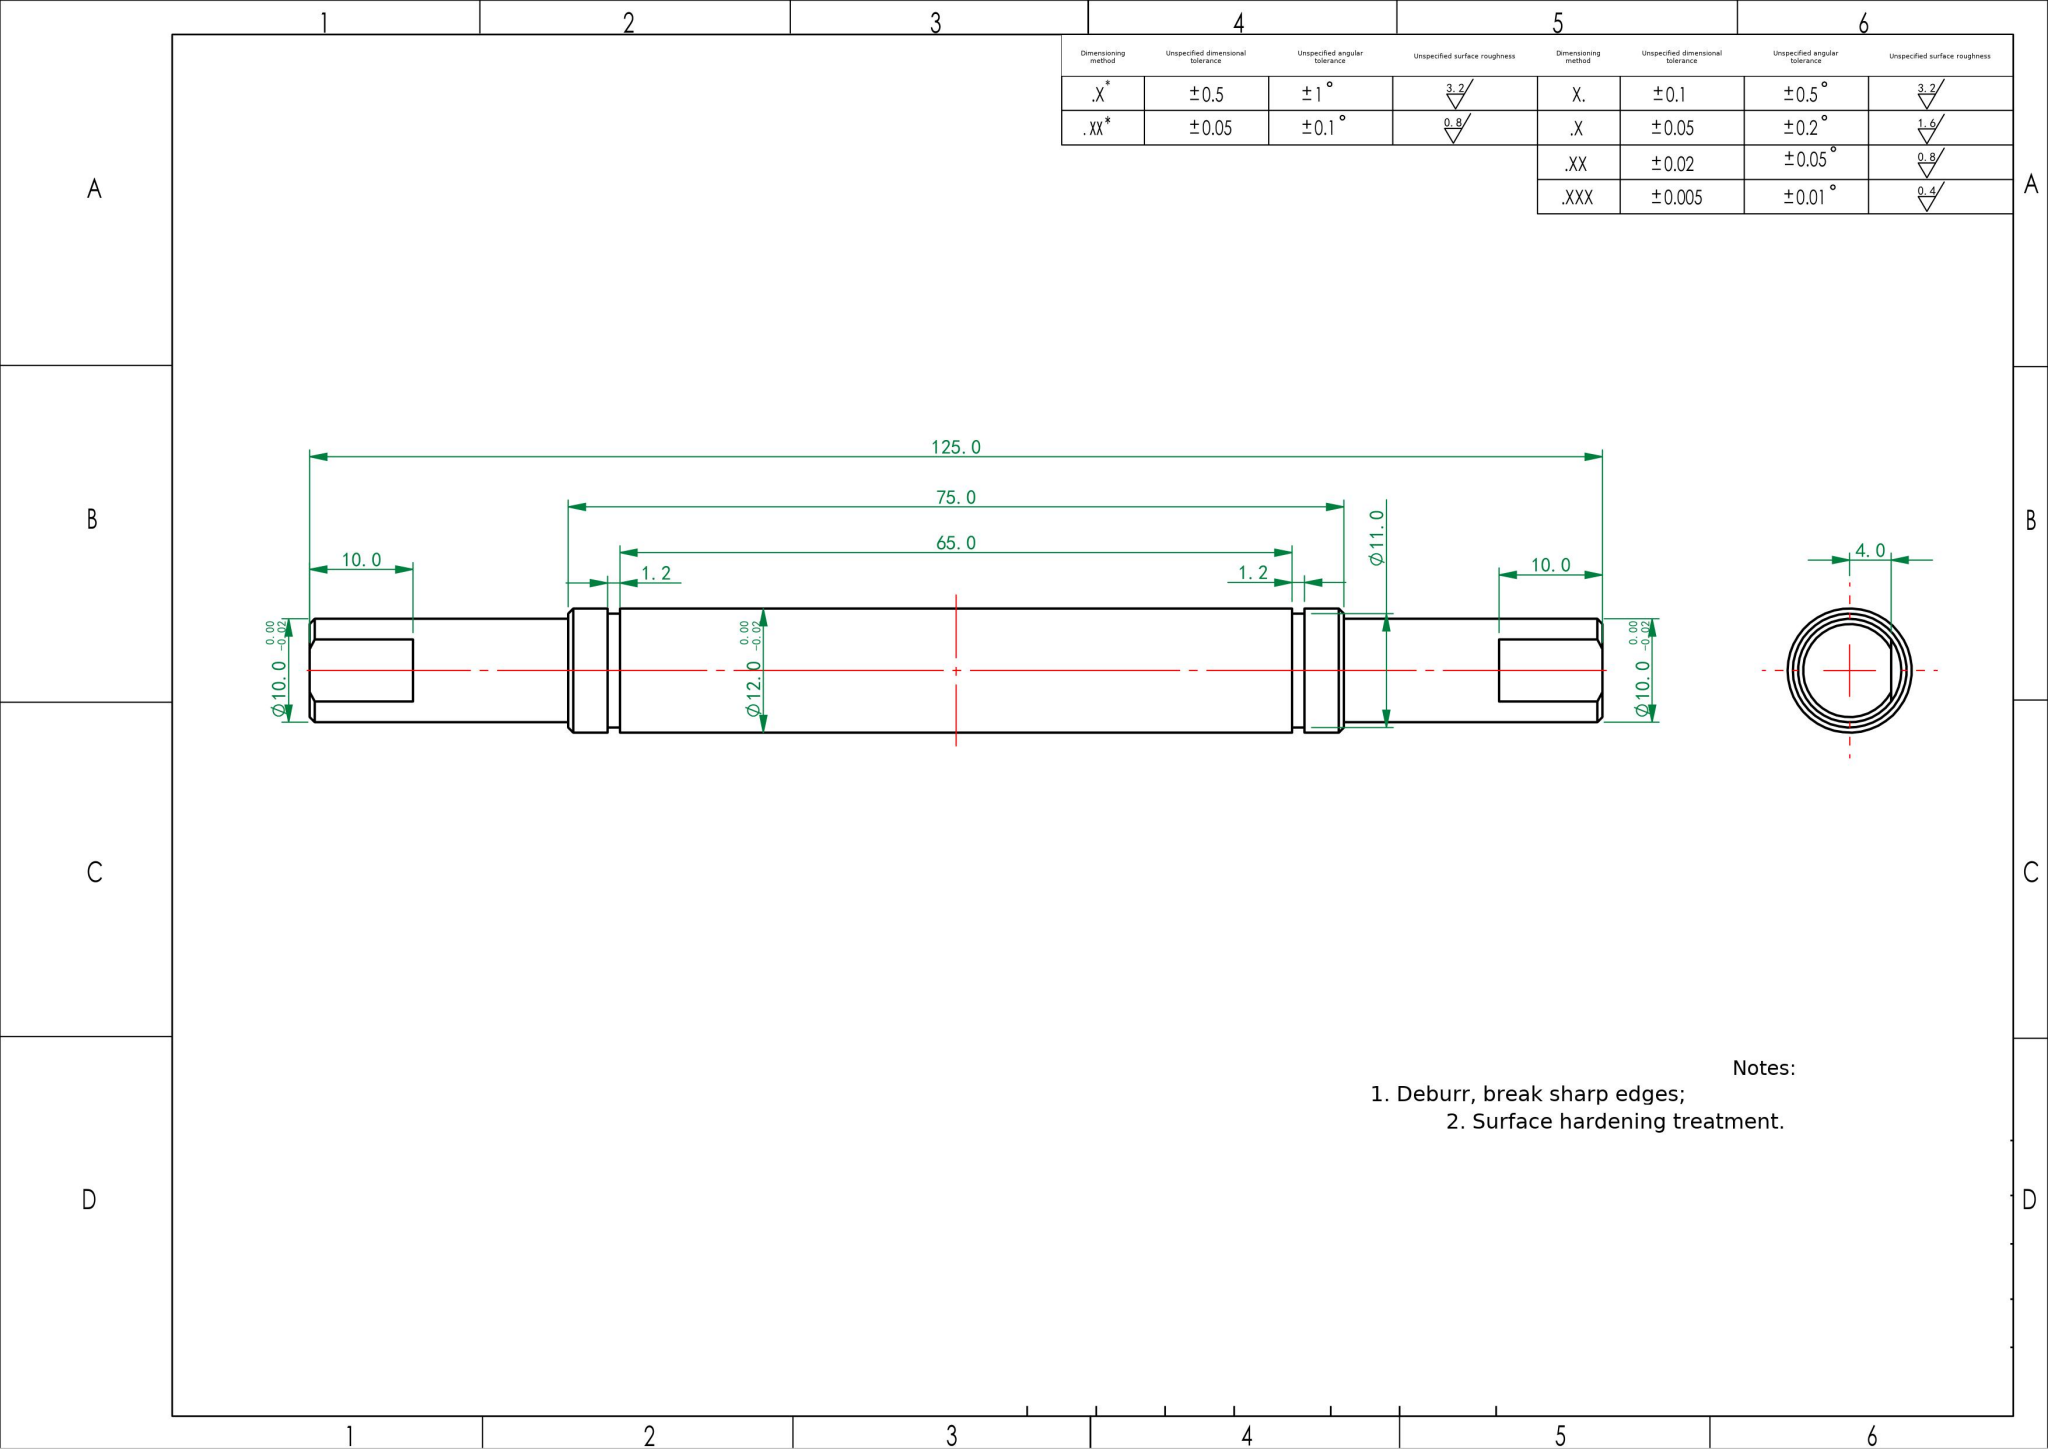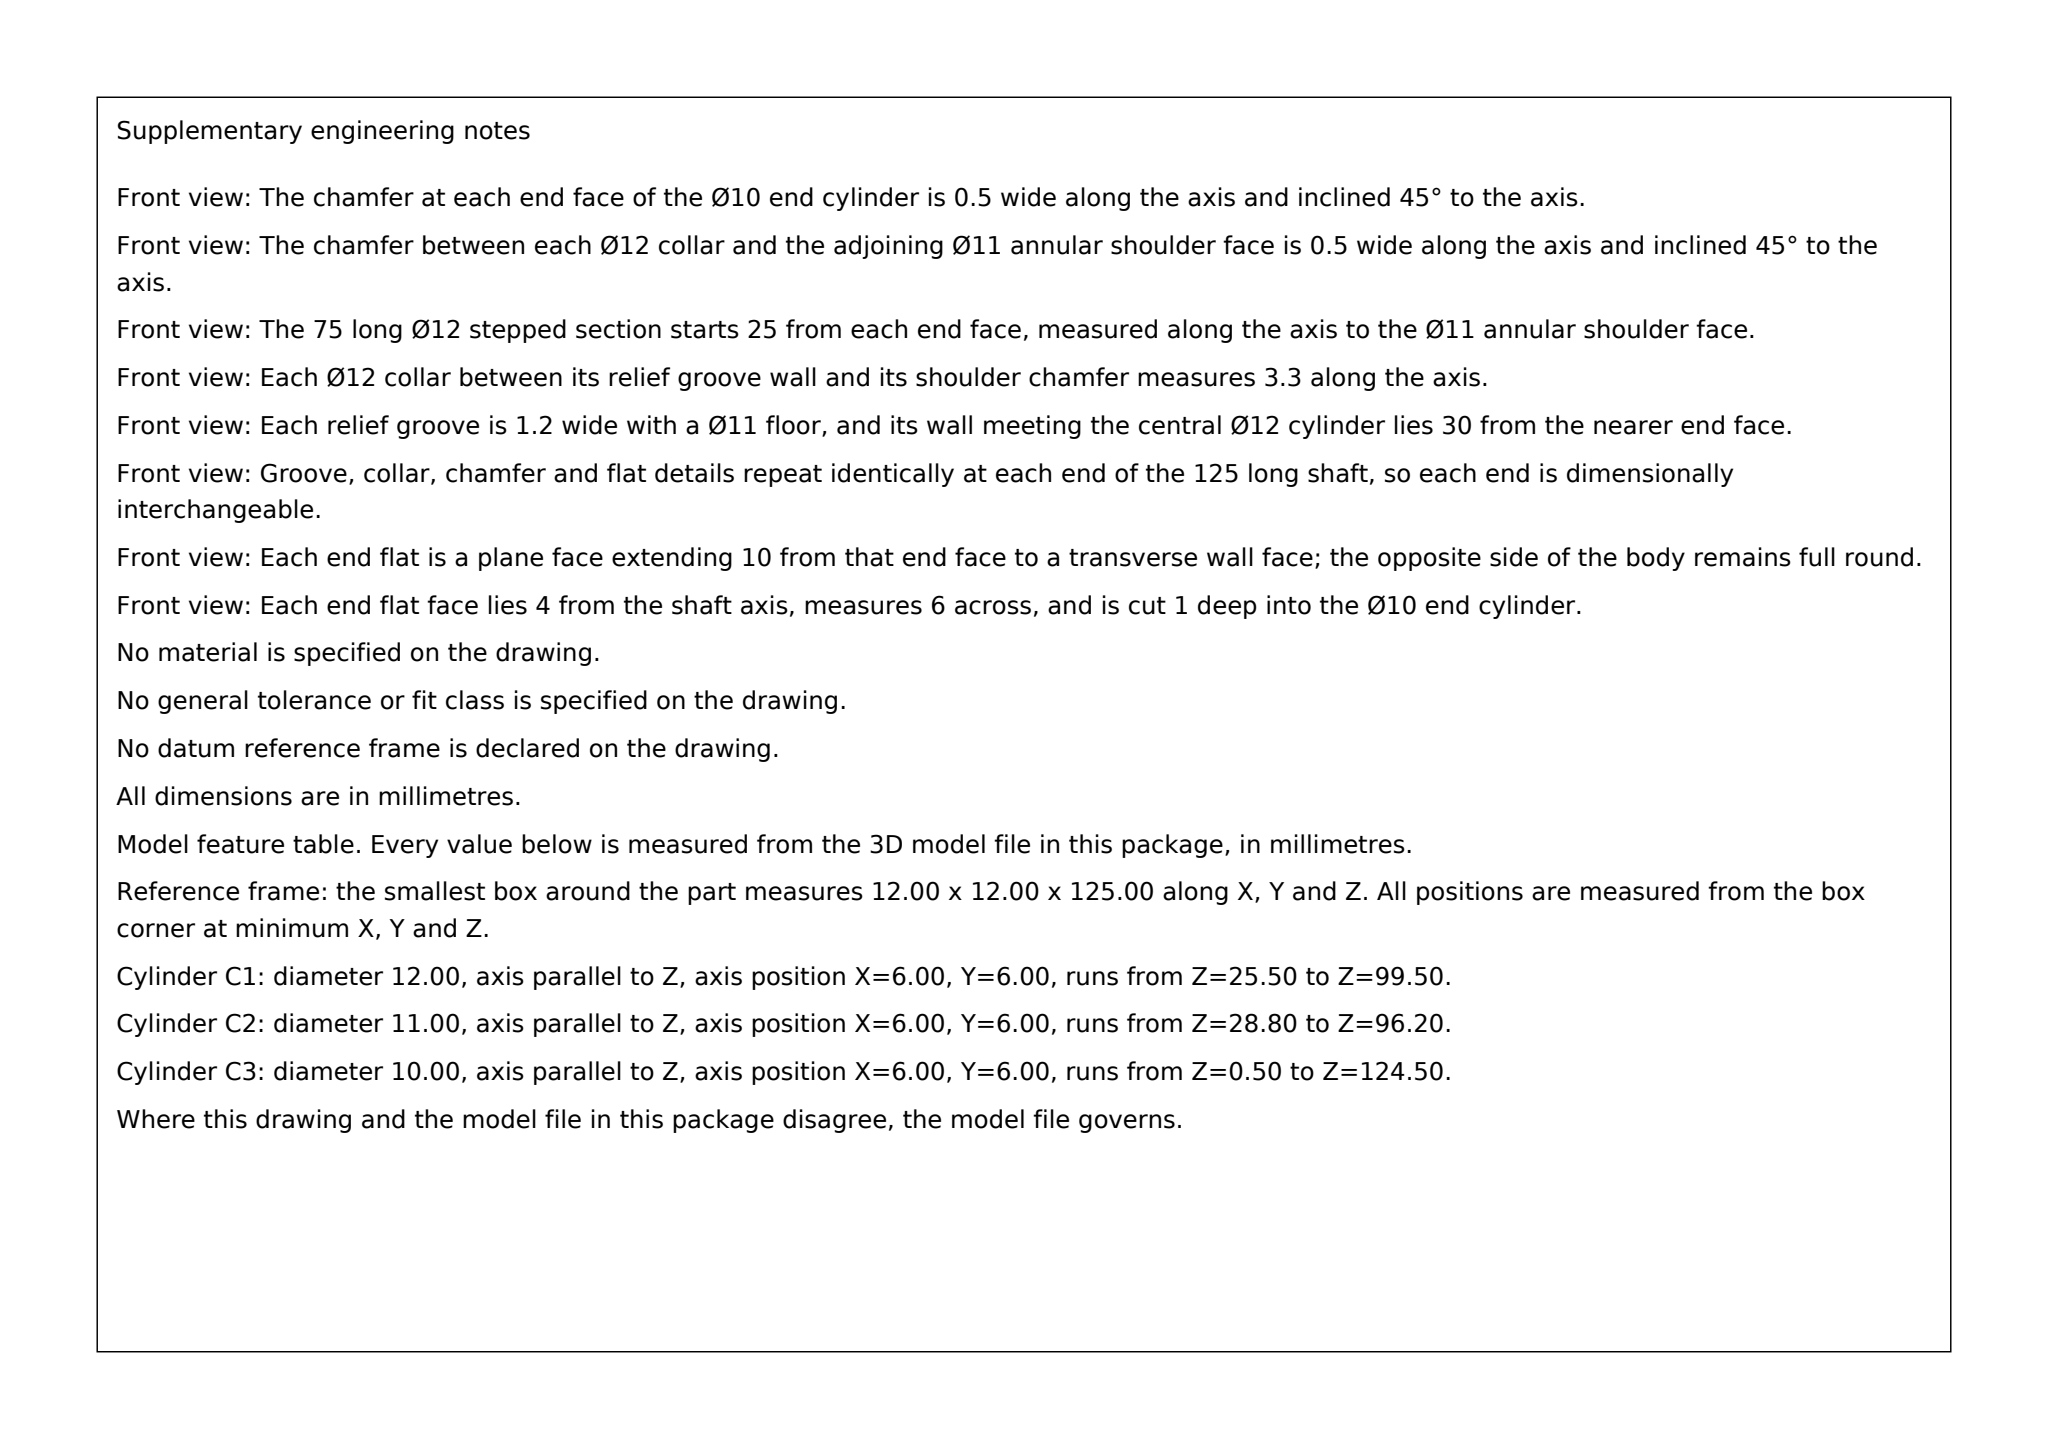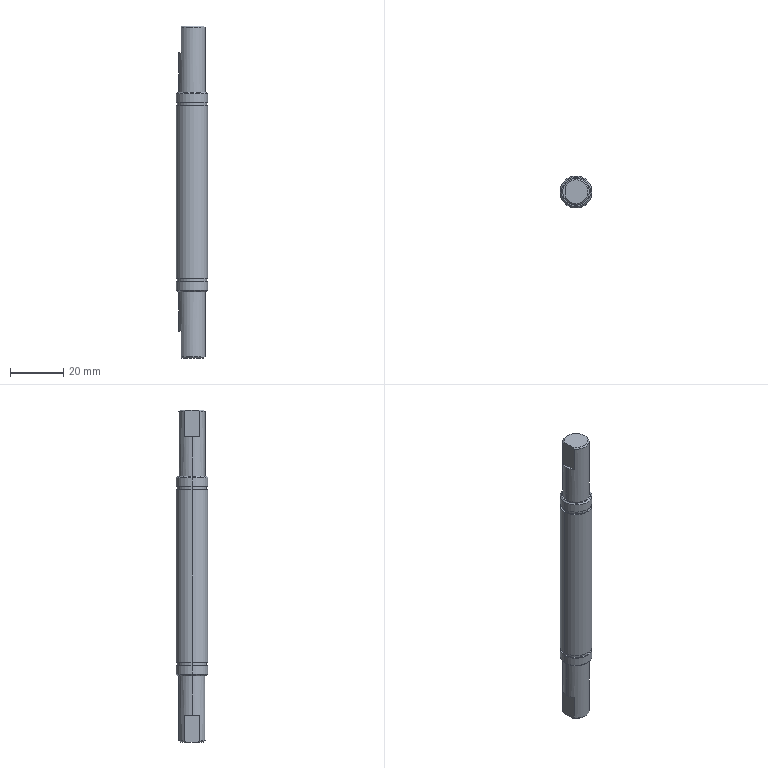Part | SolidWorks | mm | 1 solid | 33 faces | box 12 x 12 x 125 mm | volume 12269 mm3 | cylinder 14 | plane 12 | cone 7 | commonest cylinder face diameters 12 x6 11 x4 10 x4
Drawing notes:
Ø10 JOURNAL 25.0 LG EA END, FROM END FACE TO Ø12 SHOULDER | from the solid: z-planes at 0/25 and 100/125; Ø10 cyl 24.5 + C0.5 chamfer = 25.0 each end
Ø12 COLLAR 3.8 LG BETWEEN Ø10 SHOULDER AND Ø11 GROOVE, 2X | from the solid: z-planes 25.0-28.8 and 96.2-100.0; Ø12 cyl 3.3 + chamfer = 3.8
build123d program:
from build123d import *

# Parameters (mm, degrees)
SKETCH1_R           = 6
BOSS_EXTRUDE1_DEPTH = 37.5
SKETCH2_R           = 5
BOSS_EXTRUDE2_DEPTH = 25
BOSS_EXTRUDE3_START = 25
SKETCH3_R           = 5
BOSS_EXTRUDE3_DEPTH = 25
SKETCH4_W           = 0.5
SKETCH4_H           = 1.2
SKETCH5_W           = 2
SKETCH5_H           = 10
CUT_EXTRUDE1_DEPTH  = 10
CHAMFER1_SIZE       = 0.5


with BuildPart() as part:
    # Sketch1 → Boss-Extrude1 (new, symmetric)
    with BuildSketch(Plane.XY):
        Circle(SKETCH1_R)
    extrude(amount=BOSS_EXTRUDE1_DEPTH, both=True)

    # Sketch2 → Boss-Extrude2 (add)
    with BuildSketch(Plane.XY.offset(37.5)):
        Circle(SKETCH2_R)
    extrude(amount=BOSS_EXTRUDE2_DEPTH)

    # Sketch3 → Boss-Extrude3 (add)
    with BuildSketch(Plane(origin=(0, 0, -37.5), x_dir=(-1, 0, 0), z_dir=(0, 0, -1)).offset(BOSS_EXTRUDE3_START)):
        with Locations(Location((0, 0, 0), (0, 0, 180))):
            Circle(SKETCH3_R)
    extrude(amount=-BOSS_EXTRUDE3_DEPTH)

    # Sketch4 → Cut-Revolve1 (revolve, cut)
    with BuildSketch(Plane(origin=(0, 0, 0), x_dir=(1, 0, 0), z_dir=(0, 1, 0))):
        with Locations((-5.75, -33.1)):
            Rectangle(SKETCH4_W, SKETCH4_H)
        with Locations((-5.75, 33.1)):
            Rectangle(SKETCH4_W, SKETCH4_H)
    revolve(axis=Axis((0, 0, -62.5), (0, 0, 1)), mode=Mode.SUBTRACT)

    # Sketch5 → Cut-Extrude1 (cut)
    with BuildSketch(Plane.XY.offset(62.5)):
        with Locations((-5, 0)):
            Rectangle(SKETCH5_W, SKETCH5_H)
    cut_extrude1 = extrude(amount=-CUT_EXTRUDE1_DEPTH, mode=Mode.SUBTRACT)

    # Mirror1: Cut-Extrude1 across plane
    add(cut_extrude1.mirror(Plane.XY), mode=Mode.SUBTRACT)

    # Chamfer1
    chamfer1_edges = [part.edges().sort_by_distance(p)[0] for p in [
        (1.581, 4.743, -62.5),
        (-6, 0, -37.5),
        (1.581, -4.743, 62.5),
        (-6, 0, 37.5),
    ]]
    chamfer(chamfer1_edges, length=CHAMFER1_SIZE)


solid = part.part